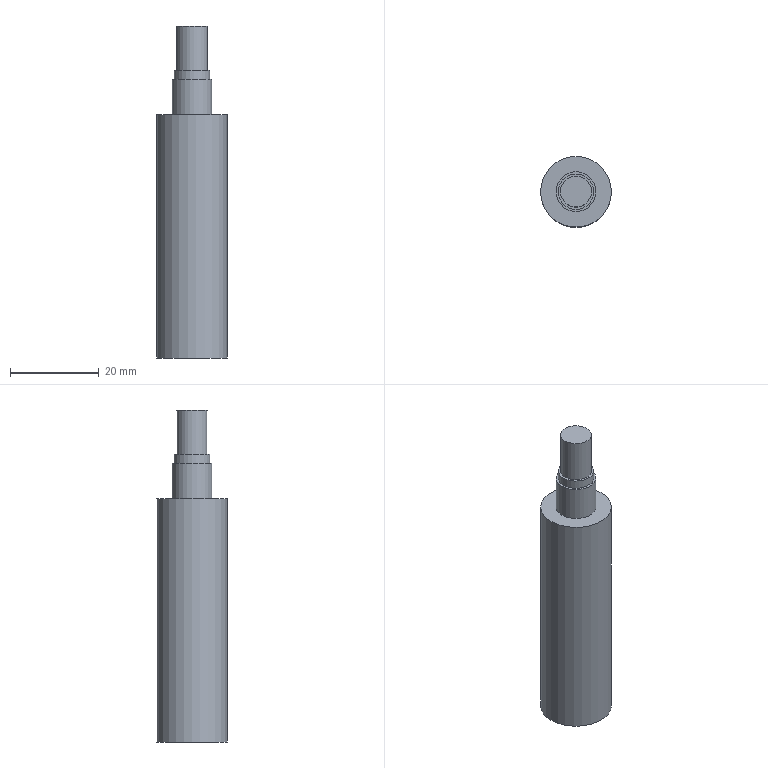Component | NX | SUPPORT_ROD | 1 solid | 11 faces | box 16 x 16 x 75 mm | volume 11719 mm3 | cylinder 5 | plane 5 | cone 1 | commonest cylinder face diameters 8 x1 16 x1 9 x1 5.795 x1 6.985 x1
STEP:
#1=CARTESIAN_POINT('',(0.,0.,0.));
#2=DIRECTION('',(0.,0.,1.));
#3=DIRECTION('',(1.,0.,0.));
#4=AXIS2_PLACEMENT_3D('',#1,#2,#3);
#5=CARTESIAN_POINT('',(4.,58.,63.));
#6=VERTEX_POINT('',#5);
#7=CARTESIAN_POINT('',(0.,58.,63.));
#8=DIRECTION('',(0.,0.,1.));
#9=DIRECTION('',(1.,0.,0.));
#10=AXIS2_PLACEMENT_3D('',#7,#8,#9);
#11=CIRCLE('',#10,4.);
#12=CARTESIAN_POINT('',(0.,58.,75.));
#13=DIRECTION('',(0.,0.,-1.));
#14=DIRECTION('',(-1.,0.,0.));
#15=AXIS2_PLACEMENT_3D('',#12,#13,#14);
#16=CYLINDRICAL_SURFACE('',#15,4.);
#17=CARTESIAN_POINT('',(9.425,12.));
#18=DIRECTION('',(-1.,0.));
#19=VECTOR('',#18,1.);
#20=LINE('',#17,#19);
#21=(GEOMETRIC_REPRESENTATION_CONTEXT(2)PARAMETRIC_REPRESENTATION_CONTEXT()REPRESENTATION_CONTEXT('',''));
#22=DEFINITIONAL_REPRESENTATION('',(#20),#21);
#23=PCURVE('',#16,#22);
#24=CARTESIAN_POINT('',(0.,58.,63.));
#25=DIRECTION('',(0.,0.,1.));
#26=DIRECTION('',(1.,0.,0.));
#27=AXIS2_PLACEMENT_3D('',#24,#25,#26);
#28=PLANE('',#27);
#29=CARTESIAN_POINT('',(0.,0.));
#30=DIRECTION('',(1.,0.));
#31=AXIS2_PLACEMENT_2D('',#29,#30);
#32=CIRCLE('',#31,4.);
#33=(GEOMETRIC_REPRESENTATION_CONTEXT(2)PARAMETRIC_REPRESENTATION_CONTEXT()REPRESENTATION_CONTEXT('',''));
#34=DEFINITIONAL_REPRESENTATION('',(#32),#33);
#35=PCURVE('',#28,#34);
#36=SURFACE_CURVE('',#11,(#23,#35),.PCURVE_S1.);
#37=EDGE_CURVE('',#6,#6,#36,.T.);
#38=ORIENTED_EDGE('',*,*,#37,.T.);
#39=CARTESIAN_POINT('',(4.,58.,65.));
#40=VERTEX_POINT('',#39);
#41=CARTESIAN_POINT('',(4.,58.,65.));
#42=CARTESIAN_POINT('',(4.,58.,63.));
#43=B_SPLINE_CURVE_WITH_KNOTS('',1,(#41,#42),.UNSPECIFIED.,.F.,.F.,(2,2),(10.,12.),.PIECEWISE_BEZIER_KNOTS.);
#44=CARTESIAN_POINT('',(3.142,0.));
#45=DIRECTION('',(0.,1.));
#46=VECTOR('',#45,1.);
#47=LINE('',#44,#46);
#48=(GEOMETRIC_REPRESENTATION_CONTEXT(2)PARAMETRIC_REPRESENTATION_CONTEXT()REPRESENTATION_CONTEXT('',''));
#49=DEFINITIONAL_REPRESENTATION('',(#47),#48);
#50=PCURVE('',#16,#49);
#51=CARTESIAN_POINT('',(9.425,0.));
#52=DIRECTION('',(0.,1.));
#53=VECTOR('',#52,1.);
#54=LINE('',#51,#53);
#55=(GEOMETRIC_REPRESENTATION_CONTEXT(2)PARAMETRIC_REPRESENTATION_CONTEXT()REPRESENTATION_CONTEXT('',''));
#56=DEFINITIONAL_REPRESENTATION('',(#54),#55);
#57=PCURVE('',#16,#56);
#58=SEAM_CURVE('',#43,(#50,#57),.PCURVE_S1.);
#59=EDGE_CURVE('',#40,#6,#58,.T.);
#60=ORIENTED_EDGE('',*,*,#59,.F.);
#61=CARTESIAN_POINT('',(0.,58.,65.));
#62=DIRECTION('',(0.,0.,1.));
#63=DIRECTION('',(1.,0.,0.));
#64=AXIS2_PLACEMENT_3D('',#61,#62,#63);
#65=CIRCLE('',#64,4.);
#66=CARTESIAN_POINT('',(9.425,10.));
#67=DIRECTION('',(-1.,0.));
#68=VECTOR('',#67,1.);
#69=LINE('',#66,#68);
#70=(GEOMETRIC_REPRESENTATION_CONTEXT(2)PARAMETRIC_REPRESENTATION_CONTEXT()REPRESENTATION_CONTEXT('',''));
#71=DEFINITIONAL_REPRESENTATION('',(#69),#70);
#72=PCURVE('',#16,#71);
#73=CARTESIAN_POINT('',(0.,58.,65.));
#74=DIRECTION('',(0.,0.,1.));
#75=DIRECTION('',(1.,0.,0.));
#76=AXIS2_PLACEMENT_3D('',#73,#74,#75);
#77=PLANE('',#76);
#78=CARTESIAN_POINT('',(0.,0.));
#79=DIRECTION('',(1.,0.));
#80=AXIS2_PLACEMENT_2D('',#78,#79);
#81=CIRCLE('',#80,4.);
#82=(GEOMETRIC_REPRESENTATION_CONTEXT(2)PARAMETRIC_REPRESENTATION_CONTEXT()REPRESENTATION_CONTEXT('',''));
#83=DEFINITIONAL_REPRESENTATION('',(#81),#82);
#84=PCURVE('',#77,#83);
#85=SURFACE_CURVE('',#65,(#72,#84),.PCURVE_S1.);
#86=EDGE_CURVE('',#40,#40,#85,.T.);
#87=ORIENTED_EDGE('',*,*,#86,.F.);
#88=ORIENTED_EDGE('',*,*,#59,.T.);
#89=EDGE_LOOP('',(#38,#60,#87,#88));
#90=FACE_BOUND('',#89,.T.);
#91=ADVANCED_FACE('',(#90),#16,.T.);
#92=CARTESIAN_POINT('',(8.,58.,55.));
#93=VERTEX_POINT('',#92);
#94=CARTESIAN_POINT('',(0.,58.,55.));
#95=DIRECTION('',(0.,0.,1.));
#96=DIRECTION('',(1.,0.,0.));
#97=AXIS2_PLACEMENT_3D('',#94,#95,#96);
#98=CIRCLE('',#97,8.);
#99=CARTESIAN_POINT('',(0.,58.,55.));
#100=DIRECTION('',(0.,0.,-1.));
#101=DIRECTION('',(-1.,0.,0.));
#102=AXIS2_PLACEMENT_3D('',#99,#100,#101);
#103=CYLINDRICAL_SURFACE('',#102,8.);
#104=CARTESIAN_POINT('',(9.425,0.));
#105=DIRECTION('',(-1.,0.));
#106=VECTOR('',#105,1.);
#107=LINE('',#104,#106);
#108=(GEOMETRIC_REPRESENTATION_CONTEXT(2)PARAMETRIC_REPRESENTATION_CONTEXT()REPRESENTATION_CONTEXT('',''));
#109=DEFINITIONAL_REPRESENTATION('',(#107),#108);
#110=PCURVE('',#103,#109);
#111=CARTESIAN_POINT('',(0.,58.,55.));
#112=DIRECTION('',(0.,0.,1.));
#113=DIRECTION('',(1.,0.,0.));
#114=AXIS2_PLACEMENT_3D('',#111,#112,#113);
#115=PLANE('',#114);
#116=CARTESIAN_POINT('',(0.,0.));
#117=DIRECTION('',(1.,0.));
#118=AXIS2_PLACEMENT_2D('',#116,#117);
#119=CIRCLE('',#118,8.);
#120=(GEOMETRIC_REPRESENTATION_CONTEXT(2)PARAMETRIC_REPRESENTATION_CONTEXT()REPRESENTATION_CONTEXT('',''));
#121=DEFINITIONAL_REPRESENTATION('',(#119),#120);
#122=PCURVE('',#115,#121);
#123=SURFACE_CURVE('',#98,(#110,#122),.PCURVE_S1.);
#124=EDGE_CURVE('',#93,#93,#123,.T.);
#125=ORIENTED_EDGE('',*,*,#124,.F.);
#126=CARTESIAN_POINT('',(8.,58.,-0.));
#127=VERTEX_POINT('',#126);
#128=CARTESIAN_POINT('',(8.,58.,55.));
#129=CARTESIAN_POINT('',(8.,58.,0.));
#130=B_SPLINE_CURVE_WITH_KNOTS('',1,(#128,#129),.UNSPECIFIED.,.F.,.F.,(2,2),(0.,55.),.PIECEWISE_BEZIER_KNOTS.);
#131=CARTESIAN_POINT('',(9.425,0.));
#132=DIRECTION('',(0.,1.));
#133=VECTOR('',#132,1.);
#134=LINE('',#131,#133);
#135=(GEOMETRIC_REPRESENTATION_CONTEXT(2)PARAMETRIC_REPRESENTATION_CONTEXT()REPRESENTATION_CONTEXT('',''));
#136=DEFINITIONAL_REPRESENTATION('',(#134),#135);
#137=PCURVE('',#103,#136);
#138=CARTESIAN_POINT('',(3.142,0.));
#139=DIRECTION('',(0.,1.));
#140=VECTOR('',#139,1.);
#141=LINE('',#138,#140);
#142=(GEOMETRIC_REPRESENTATION_CONTEXT(2)PARAMETRIC_REPRESENTATION_CONTEXT()REPRESENTATION_CONTEXT('',''));
#143=DEFINITIONAL_REPRESENTATION('',(#141),#142);
#144=PCURVE('',#103,#143);
#145=SEAM_CURVE('',#130,(#137,#144),.PCURVE_S1.);
#146=EDGE_CURVE('',#93,#127,#145,.T.);
#147=ORIENTED_EDGE('',*,*,#146,.T.);
#148=CARTESIAN_POINT('',(0.,58.,-0.));
#149=DIRECTION('',(0.,0.,1.));
#150=DIRECTION('',(1.,0.,0.));
#151=AXIS2_PLACEMENT_3D('',#148,#149,#150);
#152=CIRCLE('',#151,8.);
#153=CARTESIAN_POINT('',(9.425,55.));
#154=DIRECTION('',(-1.,0.));
#155=VECTOR('',#154,1.);
#156=LINE('',#153,#155);
#157=(GEOMETRIC_REPRESENTATION_CONTEXT(2)PARAMETRIC_REPRESENTATION_CONTEXT()REPRESENTATION_CONTEXT('',''));
#158=DEFINITIONAL_REPRESENTATION('',(#156),#157);
#159=PCURVE('',#103,#158);
#160=CARTESIAN_POINT('',(0.,58.,-0.));
#161=DIRECTION('',(0.,0.,1.));
#162=DIRECTION('',(1.,0.,0.));
#163=AXIS2_PLACEMENT_3D('',#160,#161,#162);
#164=PLANE('',#163);
#165=CARTESIAN_POINT('',(0.,0.));
#166=DIRECTION('',(1.,0.));
#167=AXIS2_PLACEMENT_2D('',#165,#166);
#168=CIRCLE('',#167,8.);
#169=(GEOMETRIC_REPRESENTATION_CONTEXT(2)PARAMETRIC_REPRESENTATION_CONTEXT()REPRESENTATION_CONTEXT('',''));
#170=DEFINITIONAL_REPRESENTATION('',(#168),#169);
#171=PCURVE('',#164,#170);
#172=SURFACE_CURVE('',#152,(#159,#171),.PCURVE_S1.);
#173=EDGE_CURVE('',#127,#127,#172,.T.);
#174=ORIENTED_EDGE('',*,*,#173,.T.);
#175=ORIENTED_EDGE('',*,*,#146,.F.);
#176=EDGE_LOOP('',(#125,#147,#174,#175));
#177=FACE_BOUND('',#176,.T.);
#178=ADVANCED_FACE('',(#177),#103,.T.);
#179=CARTESIAN_POINT('',(4.5,58.,55.));
#180=VERTEX_POINT('',#179);
#181=CARTESIAN_POINT('',(0.,58.,55.));
#182=DIRECTION('',(0.,0.,1.));
#183=DIRECTION('',(1.,0.,0.));
#184=AXIS2_PLACEMENT_3D('',#181,#182,#183);
#185=CIRCLE('',#184,4.5);
#186=CARTESIAN_POINT('',(0.,0.));
#187=DIRECTION('',(1.,0.));
#188=AXIS2_PLACEMENT_2D('',#186,#187);
#189=CIRCLE('',#188,4.5);
#190=(GEOMETRIC_REPRESENTATION_CONTEXT(2)PARAMETRIC_REPRESENTATION_CONTEXT()REPRESENTATION_CONTEXT('',''));
#191=DEFINITIONAL_REPRESENTATION('',(#189),#190);
#192=PCURVE('',#115,#191);
#193=CARTESIAN_POINT('',(0.,58.,63.));
#194=DIRECTION('',(0.,0.,-1.));
#195=DIRECTION('',(-1.,0.,0.));
#196=AXIS2_PLACEMENT_3D('',#193,#194,#195);
#197=CYLINDRICAL_SURFACE('',#196,4.5);
#198=CARTESIAN_POINT('',(9.425,8.));
#199=DIRECTION('',(-1.,0.));
#200=VECTOR('',#199,1.);
#201=LINE('',#198,#200);
#202=(GEOMETRIC_REPRESENTATION_CONTEXT(2)PARAMETRIC_REPRESENTATION_CONTEXT()REPRESENTATION_CONTEXT('',''));
#203=DEFINITIONAL_REPRESENTATION('',(#201),#202);
#204=PCURVE('',#197,#203);
#205=SURFACE_CURVE('',#185,(#192,#204),.PCURVE_S1.);
#206=EDGE_CURVE('',#180,#180,#205,.T.);
#207=ORIENTED_EDGE('',*,*,#206,.F.);
#208=EDGE_LOOP('',(#207));
#209=FACE_BOUND('',#208,.T.);
#210=ORIENTED_EDGE('',*,*,#124,.T.);
#211=EDGE_LOOP('',(#210));
#212=FACE_BOUND('',#211,.T.);
#213=ADVANCED_FACE('',(#209,#212),#115,.T.);
#214=CARTESIAN_POINT('',(2.897,58.,-0.));
#215=VERTEX_POINT('',#214);
#216=CARTESIAN_POINT('',(0.,58.,-0.));
#217=DIRECTION('',(0.,0.,1.));
#218=DIRECTION('',(1.,0.,0.));
#219=AXIS2_PLACEMENT_3D('',#216,#217,#218);
#220=CIRCLE('',#219,2.897);
#221=CARTESIAN_POINT('',(0.,0.));
#222=DIRECTION('',(1.,0.));
#223=AXIS2_PLACEMENT_2D('',#221,#222);
#224=CIRCLE('',#223,2.897);
#225=(GEOMETRIC_REPRESENTATION_CONTEXT(2)PARAMETRIC_REPRESENTATION_CONTEXT()REPRESENTATION_CONTEXT('',''));
#226=DEFINITIONAL_REPRESENTATION('',(#224),#225);
#227=PCURVE('',#164,#226);
#228=CARTESIAN_POINT('',(0.,58.,-0.));
#229=DIRECTION('',(0.,0.,1.));
#230=DIRECTION('',(1.,0.,0.));
#231=AXIS2_PLACEMENT_3D('',#228,#229,#230);
#232=CYLINDRICAL_SURFACE('',#231,2.897);
#233=CARTESIAN_POINT('',(0.,0.));
#234=DIRECTION('',(1.,0.));
#235=VECTOR('',#234,1.);
#236=LINE('',#233,#235);
#237=(GEOMETRIC_REPRESENTATION_CONTEXT(2)PARAMETRIC_REPRESENTATION_CONTEXT()REPRESENTATION_CONTEXT('',''));
#238=DEFINITIONAL_REPRESENTATION('',(#236),#237);
#239=PCURVE('',#232,#238);
#240=SURFACE_CURVE('',#220,(#227,#239),.PCURVE_S1.);
#241=EDGE_CURVE('',#215,#215,#240,.T.);
#242=ORIENTED_EDGE('',*,*,#241,.T.);
#243=EDGE_LOOP('',(#242));
#244=FACE_BOUND('',#243,.T.);
#245=ORIENTED_EDGE('',*,*,#173,.F.);
#246=EDGE_LOOP('',(#245));
#247=FACE_BOUND('',#246,.T.);
#248=ADVANCED_FACE('',(#244,#247),#164,.F.);
#249=CARTESIAN_POINT('',(4.5,58.,63.));
#250=VERTEX_POINT('',#249);
#251=CARTESIAN_POINT('',(0.,58.,63.));
#252=DIRECTION('',(0.,0.,1.));
#253=DIRECTION('',(1.,0.,0.));
#254=AXIS2_PLACEMENT_3D('',#251,#252,#253);
#255=CIRCLE('',#254,4.5);
#256=CARTESIAN_POINT('',(9.425,0.));
#257=DIRECTION('',(-1.,0.));
#258=VECTOR('',#257,1.);
#259=LINE('',#256,#258);
#260=(GEOMETRIC_REPRESENTATION_CONTEXT(2)PARAMETRIC_REPRESENTATION_CONTEXT()REPRESENTATION_CONTEXT('',''));
#261=DEFINITIONAL_REPRESENTATION('',(#259),#260);
#262=PCURVE('',#197,#261);
#263=CARTESIAN_POINT('',(0.,0.));
#264=DIRECTION('',(1.,0.));
#265=AXIS2_PLACEMENT_2D('',#263,#264);
#266=CIRCLE('',#265,4.5);
#267=(GEOMETRIC_REPRESENTATION_CONTEXT(2)PARAMETRIC_REPRESENTATION_CONTEXT()REPRESENTATION_CONTEXT('',''));
#268=DEFINITIONAL_REPRESENTATION('',(#266),#267);
#269=PCURVE('',#28,#268);
#270=SURFACE_CURVE('',#255,(#262,#269),.PCURVE_S1.);
#271=EDGE_CURVE('',#250,#250,#270,.T.);
#272=ORIENTED_EDGE('',*,*,#271,.F.);
#273=CARTESIAN_POINT('',(4.5,58.,63.));
#274=CARTESIAN_POINT('',(4.5,58.,55.));
#275=B_SPLINE_CURVE_WITH_KNOTS('',1,(#273,#274),.UNSPECIFIED.,.F.,.F.,(2,2),(0.,8.),.PIECEWISE_BEZIER_KNOTS.);
#276=CARTESIAN_POINT('',(9.425,0.));
#277=DIRECTION('',(0.,1.));
#278=VECTOR('',#277,1.);
#279=LINE('',#276,#278);
#280=(GEOMETRIC_REPRESENTATION_CONTEXT(2)PARAMETRIC_REPRESENTATION_CONTEXT()REPRESENTATION_CONTEXT('',''));
#281=DEFINITIONAL_REPRESENTATION('',(#279),#280);
#282=PCURVE('',#197,#281);
#283=CARTESIAN_POINT('',(3.142,0.));
#284=DIRECTION('',(0.,1.));
#285=VECTOR('',#284,1.);
#286=LINE('',#283,#285);
#287=(GEOMETRIC_REPRESENTATION_CONTEXT(2)PARAMETRIC_REPRESENTATION_CONTEXT()REPRESENTATION_CONTEXT('',''));
#288=DEFINITIONAL_REPRESENTATION('',(#286),#287);
#289=PCURVE('',#197,#288);
#290=SEAM_CURVE('',#275,(#282,#289),.PCURVE_S1.);
#291=EDGE_CURVE('',#250,#180,#290,.T.);
#292=ORIENTED_EDGE('',*,*,#291,.T.);
#293=ORIENTED_EDGE('',*,*,#206,.T.);
#294=ORIENTED_EDGE('',*,*,#291,.F.);
#295=EDGE_LOOP('',(#272,#292,#293,#294));
#296=FACE_BOUND('',#295,.T.);
#297=ADVANCED_FACE('',(#296),#197,.T.);
#298=ORIENTED_EDGE('',*,*,#37,.F.);
#299=EDGE_LOOP('',(#298));
#300=FACE_BOUND('',#299,.T.);
#301=ORIENTED_EDGE('',*,*,#271,.T.);
#302=EDGE_LOOP('',(#301));
#303=FACE_BOUND('',#302,.T.);
#304=ADVANCED_FACE('',(#300,#303),#28,.T.);
#305=CARTESIAN_POINT('',(-2.897,58.,12.));
#306=VERTEX_POINT('',#305);
#307=CARTESIAN_POINT('',(2.897,58.,12.));
#308=VERTEX_POINT('',#307);
#309=CARTESIAN_POINT('',(0.,58.,12.));
#310=DIRECTION('',(0.,0.,-1.));
#311=DIRECTION('',(1.,0.,0.));
#312=AXIS2_PLACEMENT_3D('',#309,#310,#311);
#313=CIRCLE('',#312,2.897);
#314=CARTESIAN_POINT('',(0.,58.,12.));
#315=DIRECTION('',(0.,0.,-1.));
#316=DIRECTION('',(-1.,0.,0.));
#317=AXIS2_PLACEMENT_3D('',#314,#315,#316);
#318=CONICAL_SURFACE('',#317,2.897,1.03);
#319=CARTESIAN_POINT('',(-3.142,0.));
#320=DIRECTION('',(1.,0.));
#321=VECTOR('',#320,1.);
#322=LINE('',#319,#321);
#323=(GEOMETRIC_REPRESENTATION_CONTEXT(2)PARAMETRIC_REPRESENTATION_CONTEXT()REPRESENTATION_CONTEXT('',''));
#324=DEFINITIONAL_REPRESENTATION('',(#322),#323);
#325=PCURVE('',#318,#324);
#326=CARTESIAN_POINT('',(6.283,12.));
#327=DIRECTION('',(-1.,0.));
#328=VECTOR('',#327,1.);
#329=LINE('',#326,#328);
#330=(GEOMETRIC_REPRESENTATION_CONTEXT(2)PARAMETRIC_REPRESENTATION_CONTEXT()REPRESENTATION_CONTEXT('',''));
#331=DEFINITIONAL_REPRESENTATION('',(#329),#330);
#332=PCURVE('',#232,#331);
#333=SURFACE_CURVE('',#313,(#325,#332),.PCURVE_S1.);
#334=EDGE_CURVE('',#306,#308,#333,.T.);
#335=ORIENTED_EDGE('',*,*,#334,.F.);
#336=CARTESIAN_POINT('',(0.,58.,13.741));
#337=VERTEX_POINT('',#336);
#338=CARTESIAN_POINT('',(0.,58.,13.741));
#339=CARTESIAN_POINT('',(-2.897,58.,12.));
#340=B_SPLINE_CURVE_WITH_KNOTS('',1,(#338,#339),.UNSPECIFIED.,.F.,.F.,(2,2),(-3.38,0.),.PIECEWISE_BEZIER_KNOTS.);
#341=CARTESIAN_POINT('',(0.,0.));
#342=DIRECTION('',(0.,1.));
#343=VECTOR('',#342,1.);
#344=LINE('',#341,#343);
#345=(GEOMETRIC_REPRESENTATION_CONTEXT(2)PARAMETRIC_REPRESENTATION_CONTEXT()REPRESENTATION_CONTEXT('',''));
#346=DEFINITIONAL_REPRESENTATION('',(#344),#345);
#347=PCURVE('',#318,#346);
#348=CARTESIAN_POINT('',(6.283,0.));
#349=DIRECTION('',(0.,1.));
#350=VECTOR('',#349,1.);
#351=LINE('',#348,#350);
#352=(GEOMETRIC_REPRESENTATION_CONTEXT(2)PARAMETRIC_REPRESENTATION_CONTEXT()REPRESENTATION_CONTEXT('',''));
#353=DEFINITIONAL_REPRESENTATION('',(#351),#352);
#354=PCURVE('',#318,#353);
#355=SEAM_CURVE('',#340,(#347,#354),.PCURVE_S1.);
#356=EDGE_CURVE('',#337,#306,#355,.T.);
#357=ORIENTED_EDGE('',*,*,#356,.F.);
#358=ORIENTED_EDGE('',*,*,#356,.T.);
#359=CARTESIAN_POINT('',(0.,58.,12.));
#360=DIRECTION('',(0.,0.,-1.));
#361=DIRECTION('',(1.,0.,0.));
#362=AXIS2_PLACEMENT_3D('',#359,#360,#361);
#363=CIRCLE('',#362,2.897);
#364=CARTESIAN_POINT('',(3.142,0.));
#365=DIRECTION('',(1.,0.));
#366=VECTOR('',#365,1.);
#367=LINE('',#364,#366);
#368=(GEOMETRIC_REPRESENTATION_CONTEXT(2)PARAMETRIC_REPRESENTATION_CONTEXT()REPRESENTATION_CONTEXT('',''));
#369=DEFINITIONAL_REPRESENTATION('',(#367),#368);
#370=PCURVE('',#318,#369);
#371=CARTESIAN_POINT('',(6.283,12.));
#372=DIRECTION('',(-1.,0.));
#373=VECTOR('',#372,1.);
#374=LINE('',#371,#373);
#375=(GEOMETRIC_REPRESENTATION_CONTEXT(2)PARAMETRIC_REPRESENTATION_CONTEXT()REPRESENTATION_CONTEXT('',''));
#376=DEFINITIONAL_REPRESENTATION('',(#374),#375);
#377=PCURVE('',#232,#376);
#378=SURFACE_CURVE('',#363,(#370,#377),.PCURVE_S1.);
#379=EDGE_CURVE('',#308,#306,#378,.T.);
#380=ORIENTED_EDGE('',*,*,#379,.F.);
#381=EDGE_LOOP('',(#335,#357,#358,#380));
#382=FACE_BOUND('',#381,.F.);
#383=ADVANCED_FACE('',(#382),#318,.F.);
#384=ORIENTED_EDGE('',*,*,#334,.T.);
#385=CARTESIAN_POINT('',(2.897,58.,-0.));
#386=CARTESIAN_POINT('',(2.897,58.,12.));
#387=B_SPLINE_CURVE_WITH_KNOTS('',1,(#385,#386),.UNSPECIFIED.,.F.,.F.,(2,2),(0.,12.),.PIECEWISE_BEZIER_KNOTS.);
#388=CARTESIAN_POINT('',(0.,0.));
#389=DIRECTION('',(0.,1.));
#390=VECTOR('',#389,1.);
#391=LINE('',#388,#390);
#392=(GEOMETRIC_REPRESENTATION_CONTEXT(2)PARAMETRIC_REPRESENTATION_CONTEXT()REPRESENTATION_CONTEXT('',''));
#393=DEFINITIONAL_REPRESENTATION('',(#391),#392);
#394=PCURVE('',#232,#393);
#395=CARTESIAN_POINT('',(6.283,0.));
#396=DIRECTION('',(0.,1.));
#397=VECTOR('',#396,1.);
#398=LINE('',#395,#397);
#399=(GEOMETRIC_REPRESENTATION_CONTEXT(2)PARAMETRIC_REPRESENTATION_CONTEXT()REPRESENTATION_CONTEXT('',''));
#400=DEFINITIONAL_REPRESENTATION('',(#398),#399);
#401=PCURVE('',#232,#400);
#402=SEAM_CURVE('',#387,(#394,#401),.PCURVE_S1.);
#403=EDGE_CURVE('',#215,#308,#402,.T.);
#404=ORIENTED_EDGE('',*,*,#403,.F.);
#405=ORIENTED_EDGE('',*,*,#241,.T.);
#406=ORIENTED_EDGE('',*,*,#403,.T.);
#407=ORIENTED_EDGE('',*,*,#379,.T.);
#408=EDGE_LOOP('',(#384,#404,#405,#406,#407));
#409=FACE_BOUND('',#408,.F.);
#410=ADVANCED_FACE('',(#409),#232,.F.);
#411=CARTESIAN_POINT('',(3.493,58.,65.));
#412=VERTEX_POINT('',#411);
#413=CARTESIAN_POINT('',(0.,58.,65.));
#414=DIRECTION('',(0.,0.,-1.));
#415=DIRECTION('',(1.,0.,0.));
#416=AXIS2_PLACEMENT_3D('',#413,#414,#415);
#417=CIRCLE('',#416,3.493);
#418=CARTESIAN_POINT('',(3.493,0.));
#419=CARTESIAN_POINT('',(3.493,-6.049));
#420=CARTESIAN_POINT('',(-1.746,-3.025));
#421=CARTESIAN_POINT('',(-6.985,-0.));
#422=CARTESIAN_POINT('',(-1.746,3.025));
#423=CARTESIAN_POINT('',(3.493,6.049));
#424=CARTESIAN_POINT('',(3.493,0.));
#425=(BOUNDED_CURVE()B_SPLINE_CURVE(2,(#418,#419,#420,#421,#422,#423,#424),.UNSPECIFIED.,.T.,.F.)B_SPLINE_CURVE_WITH_KNOTS((1,2,2,2,2,1),(-2.094,0.,2.094,4.189,6.283,8.378),.UNSPECIFIED.)CURVE()GEOMETRIC_REPRESENTATION_ITEM()RATIONAL_B_SPLINE_CURVE((1.,0.5,1.,0.5,1.,0.5,1.))REPRESENTATION_ITEM(''));
#426=(GEOMETRIC_REPRESENTATION_CONTEXT(2)PARAMETRIC_REPRESENTATION_CONTEXT()REPRESENTATION_CONTEXT('',''));
#427=DEFINITIONAL_REPRESENTATION('',(#425),#426);
#428=PCURVE('',#77,#427);
#429=CARTESIAN_POINT('',(0.,58.,76.));
#430=DIRECTION('',(0.,0.,-1.));
#431=DIRECTION('',(-1.,0.,0.));
#432=AXIS2_PLACEMENT_3D('',#429,#430,#431);
#433=CYLINDRICAL_SURFACE('',#432,3.493);
#434=CARTESIAN_POINT('',(3.142,11.));
#435=DIRECTION('',(1.,0.));
#436=VECTOR('',#435,1.);
#437=LINE('',#434,#436);
#438=(GEOMETRIC_REPRESENTATION_CONTEXT(2)PARAMETRIC_REPRESENTATION_CONTEXT()REPRESENTATION_CONTEXT('',''));
#439=DEFINITIONAL_REPRESENTATION('',(#437),#438);
#440=PCURVE('',#433,#439);
#441=SURFACE_CURVE('',#417,(#428,#440),.PCURVE_S1.);
#442=EDGE_CURVE('',#412,#412,#441,.T.);
#443=ORIENTED_EDGE('',*,*,#442,.T.);
#444=EDGE_LOOP('',(#443));
#445=FACE_BOUND('',#444,.T.);
#446=ORIENTED_EDGE('',*,*,#86,.T.);
#447=EDGE_LOOP('',(#446));
#448=FACE_BOUND('',#447,.T.);
#449=ADVANCED_FACE('',(#445,#448),#77,.T.);
#450=CARTESIAN_POINT('',(3.493,58.,75.));
#451=VERTEX_POINT('',#450);
#452=CARTESIAN_POINT('',(0.,58.,75.));
#453=DIRECTION('',(0.,0.,-1.));
#454=DIRECTION('',(1.,0.,0.));
#455=AXIS2_PLACEMENT_3D('',#452,#453,#454);
#456=CIRCLE('',#455,3.493);
#457=CARTESIAN_POINT('',(3.142,1.));
#458=DIRECTION('',(1.,0.));
#459=VECTOR('',#458,1.);
#460=LINE('',#457,#459);
#461=(GEOMETRIC_REPRESENTATION_CONTEXT(2)PARAMETRIC_REPRESENTATION_CONTEXT()REPRESENTATION_CONTEXT('',''));
#462=DEFINITIONAL_REPRESENTATION('',(#460),#461);
#463=PCURVE('',#433,#462);
#464=CARTESIAN_POINT('',(0.,58.,75.));
#465=DIRECTION('',(0.,0.,1.));
#466=DIRECTION('',(1.,0.,0.));
#467=AXIS2_PLACEMENT_3D('',#464,#465,#466);
#468=PLANE('',#467);
#469=CARTESIAN_POINT('',(3.493,0.));
#470=CARTESIAN_POINT('',(3.493,-6.049));
#471=CARTESIAN_POINT('',(-1.746,-3.025));
#472=CARTESIAN_POINT('',(-6.985,-0.));
#473=CARTESIAN_POINT('',(-1.746,3.025));
#474=CARTESIAN_POINT('',(3.493,6.049));
#475=CARTESIAN_POINT('',(3.493,0.));
#476=(BOUNDED_CURVE()B_SPLINE_CURVE(2,(#469,#470,#471,#472,#473,#474,#475),.UNSPECIFIED.,.T.,.F.)B_SPLINE_CURVE_WITH_KNOTS((1,2,2,2,2,1),(-2.094,0.,2.094,4.189,6.283,8.378),.UNSPECIFIED.)CURVE()GEOMETRIC_REPRESENTATION_ITEM()RATIONAL_B_SPLINE_CURVE((1.,0.5,1.,0.5,1.,0.5,1.))REPRESENTATION_ITEM(''));
#477=(GEOMETRIC_REPRESENTATION_CONTEXT(2)PARAMETRIC_REPRESENTATION_CONTEXT()REPRESENTATION_CONTEXT('',''));
#478=DEFINITIONAL_REPRESENTATION('',(#476),#477);
#479=PCURVE('',#468,#478);
#480=SURFACE_CURVE('',#456,(#463,#479),.PCURVE_S1.);
#481=EDGE_CURVE('',#451,#451,#480,.T.);
#482=ORIENTED_EDGE('',*,*,#481,.T.);
#483=CARTESIAN_POINT('',(3.493,58.,75.));
#484=CARTESIAN_POINT('',(3.493,58.,65.));
#485=B_SPLINE_CURVE_WITH_KNOTS('',1,(#483,#484),.UNSPECIFIED.,.F.,.F.,(2,2),(1.,11.),.PIECEWISE_BEZIER_KNOTS.);
#486=CARTESIAN_POINT('',(9.425,0.));
#487=DIRECTION('',(0.,1.));
#488=VECTOR('',#487,1.);
#489=LINE('',#486,#488);
#490=(GEOMETRIC_REPRESENTATION_CONTEXT(2)PARAMETRIC_REPRESENTATION_CONTEXT()REPRESENTATION_CONTEXT('',''));
#491=DEFINITIONAL_REPRESENTATION('',(#489),#490);
#492=PCURVE('',#433,#491);
#493=CARTESIAN_POINT('',(3.142,0.));
#494=DIRECTION('',(0.,1.));
#495=VECTOR('',#494,1.);
#496=LINE('',#493,#495);
#497=(GEOMETRIC_REPRESENTATION_CONTEXT(2)PARAMETRIC_REPRESENTATION_CONTEXT()REPRESENTATION_CONTEXT('',''));
#498=DEFINITIONAL_REPRESENTATION('',(#496),#497);
#499=PCURVE('',#433,#498);
#500=SEAM_CURVE('',#485,(#492,#499),.PCURVE_S1.);
#501=EDGE_CURVE('',#451,#412,#500,.T.);
#502=ORIENTED_EDGE('',*,*,#501,.T.);
#503=ORIENTED_EDGE('',*,*,#442,.F.);
#504=ORIENTED_EDGE('',*,*,#501,.F.);
#505=EDGE_LOOP('',(#482,#502,#503,#504));
#506=FACE_BOUND('',#505,.T.);
#507=ADVANCED_FACE('',(#506),#433,.T.);
#508=ORIENTED_EDGE('',*,*,#481,.F.);
#509=EDGE_LOOP('',(#508));
#510=FACE_BOUND('',#509,.T.);
#511=ADVANCED_FACE('',(#510),#468,.T.);
#512=CLOSED_SHELL('',(#91,#178,#213,#248,#297,#304,#383,#410,#449,#507,#511));
#513=MANIFOLD_SOLID_BREP('',#512);
#514=(LENGTH_UNIT()NAMED_UNIT(*)SI_UNIT(.MILLI.,.METRE.));
#515=UNCERTAINTY_MEASURE_WITH_UNIT(LENGTH_MEASURE(0.00001),#514,'','');
#516=(NAMED_UNIT(*)PLANE_ANGLE_UNIT()SI_UNIT($,.RADIAN.));
#517=(NAMED_UNIT(*)SI_UNIT($,.STERADIAN.)SOLID_ANGLE_UNIT());
#518=(GEOMETRIC_REPRESENTATION_CONTEXT(3)GLOBAL_UNCERTAINTY_ASSIGNED_CONTEXT((#515))GLOBAL_UNIT_ASSIGNED_CONTEXT((#514,#516,#517))REPRESENTATION_CONTEXT('',''));
#519=ADVANCED_BREP_SHAPE_REPRESENTATION('',(#4,#513),#518);